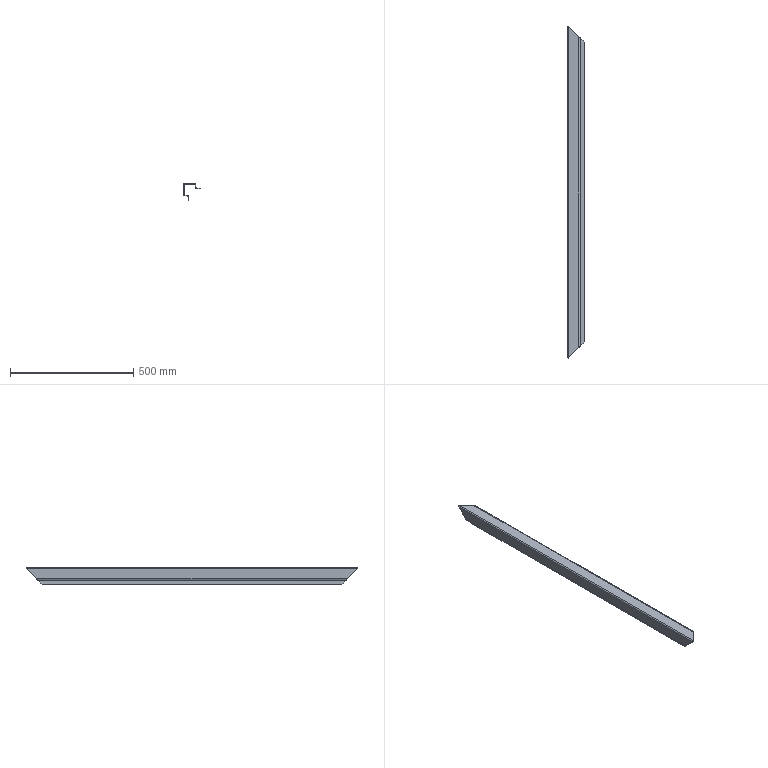Component | SolidWorks | BoxWelding-1_SupportPlate1-2 | 1 solid | 48 faces | volume 416933 mm3 | plane 26 | spline 12 | cylinder 10 | commonest cylinder face diameters 8 x5 4 x5